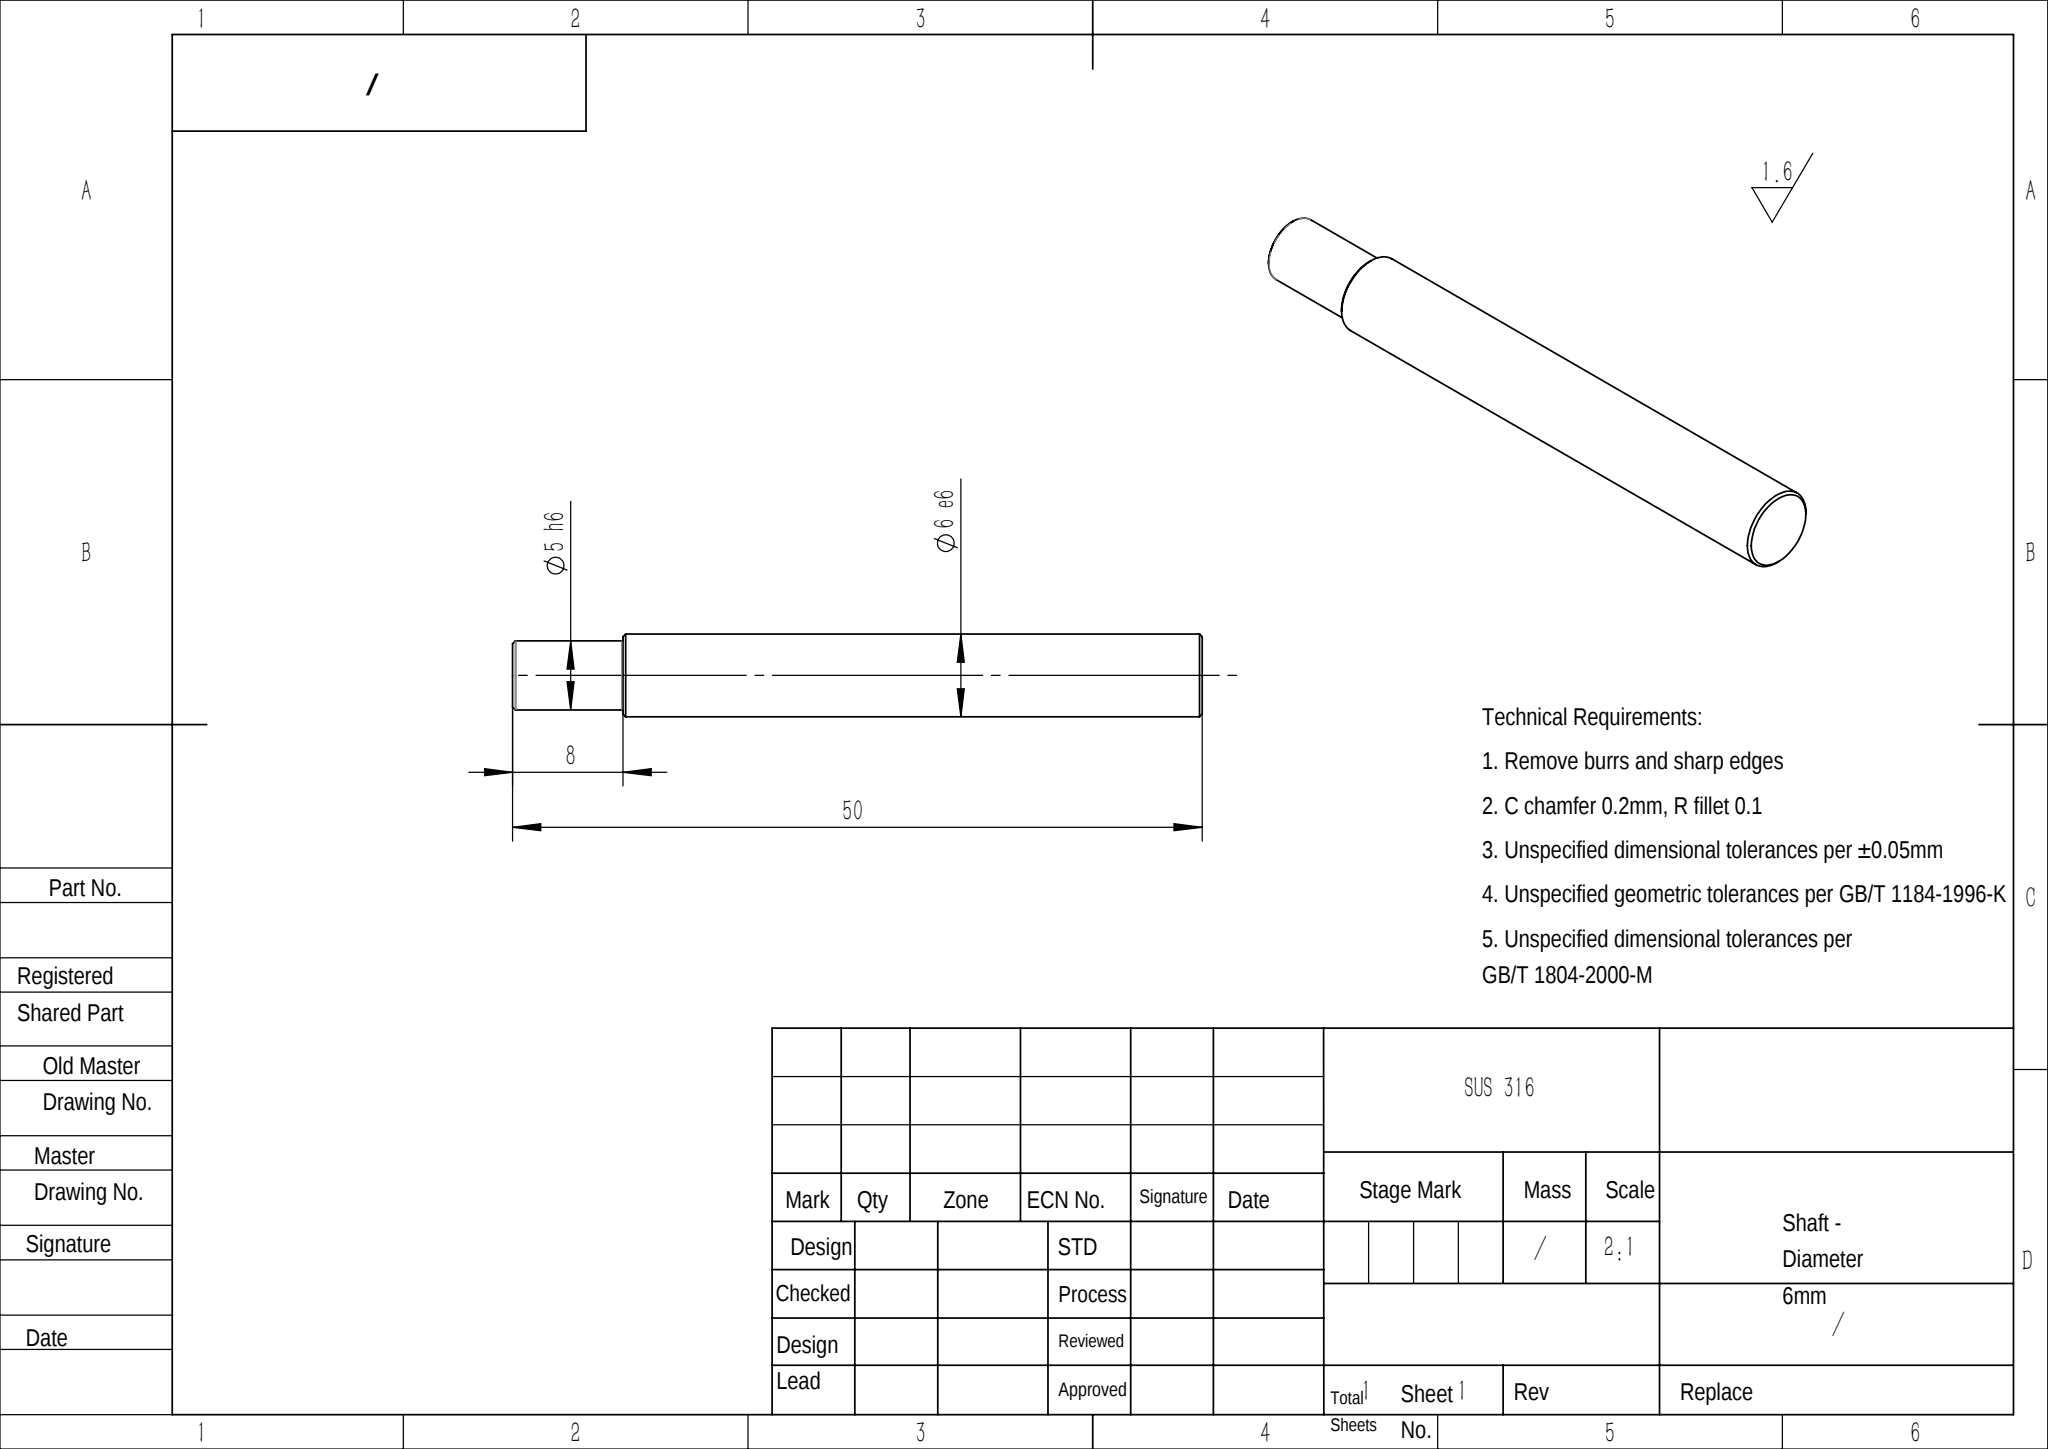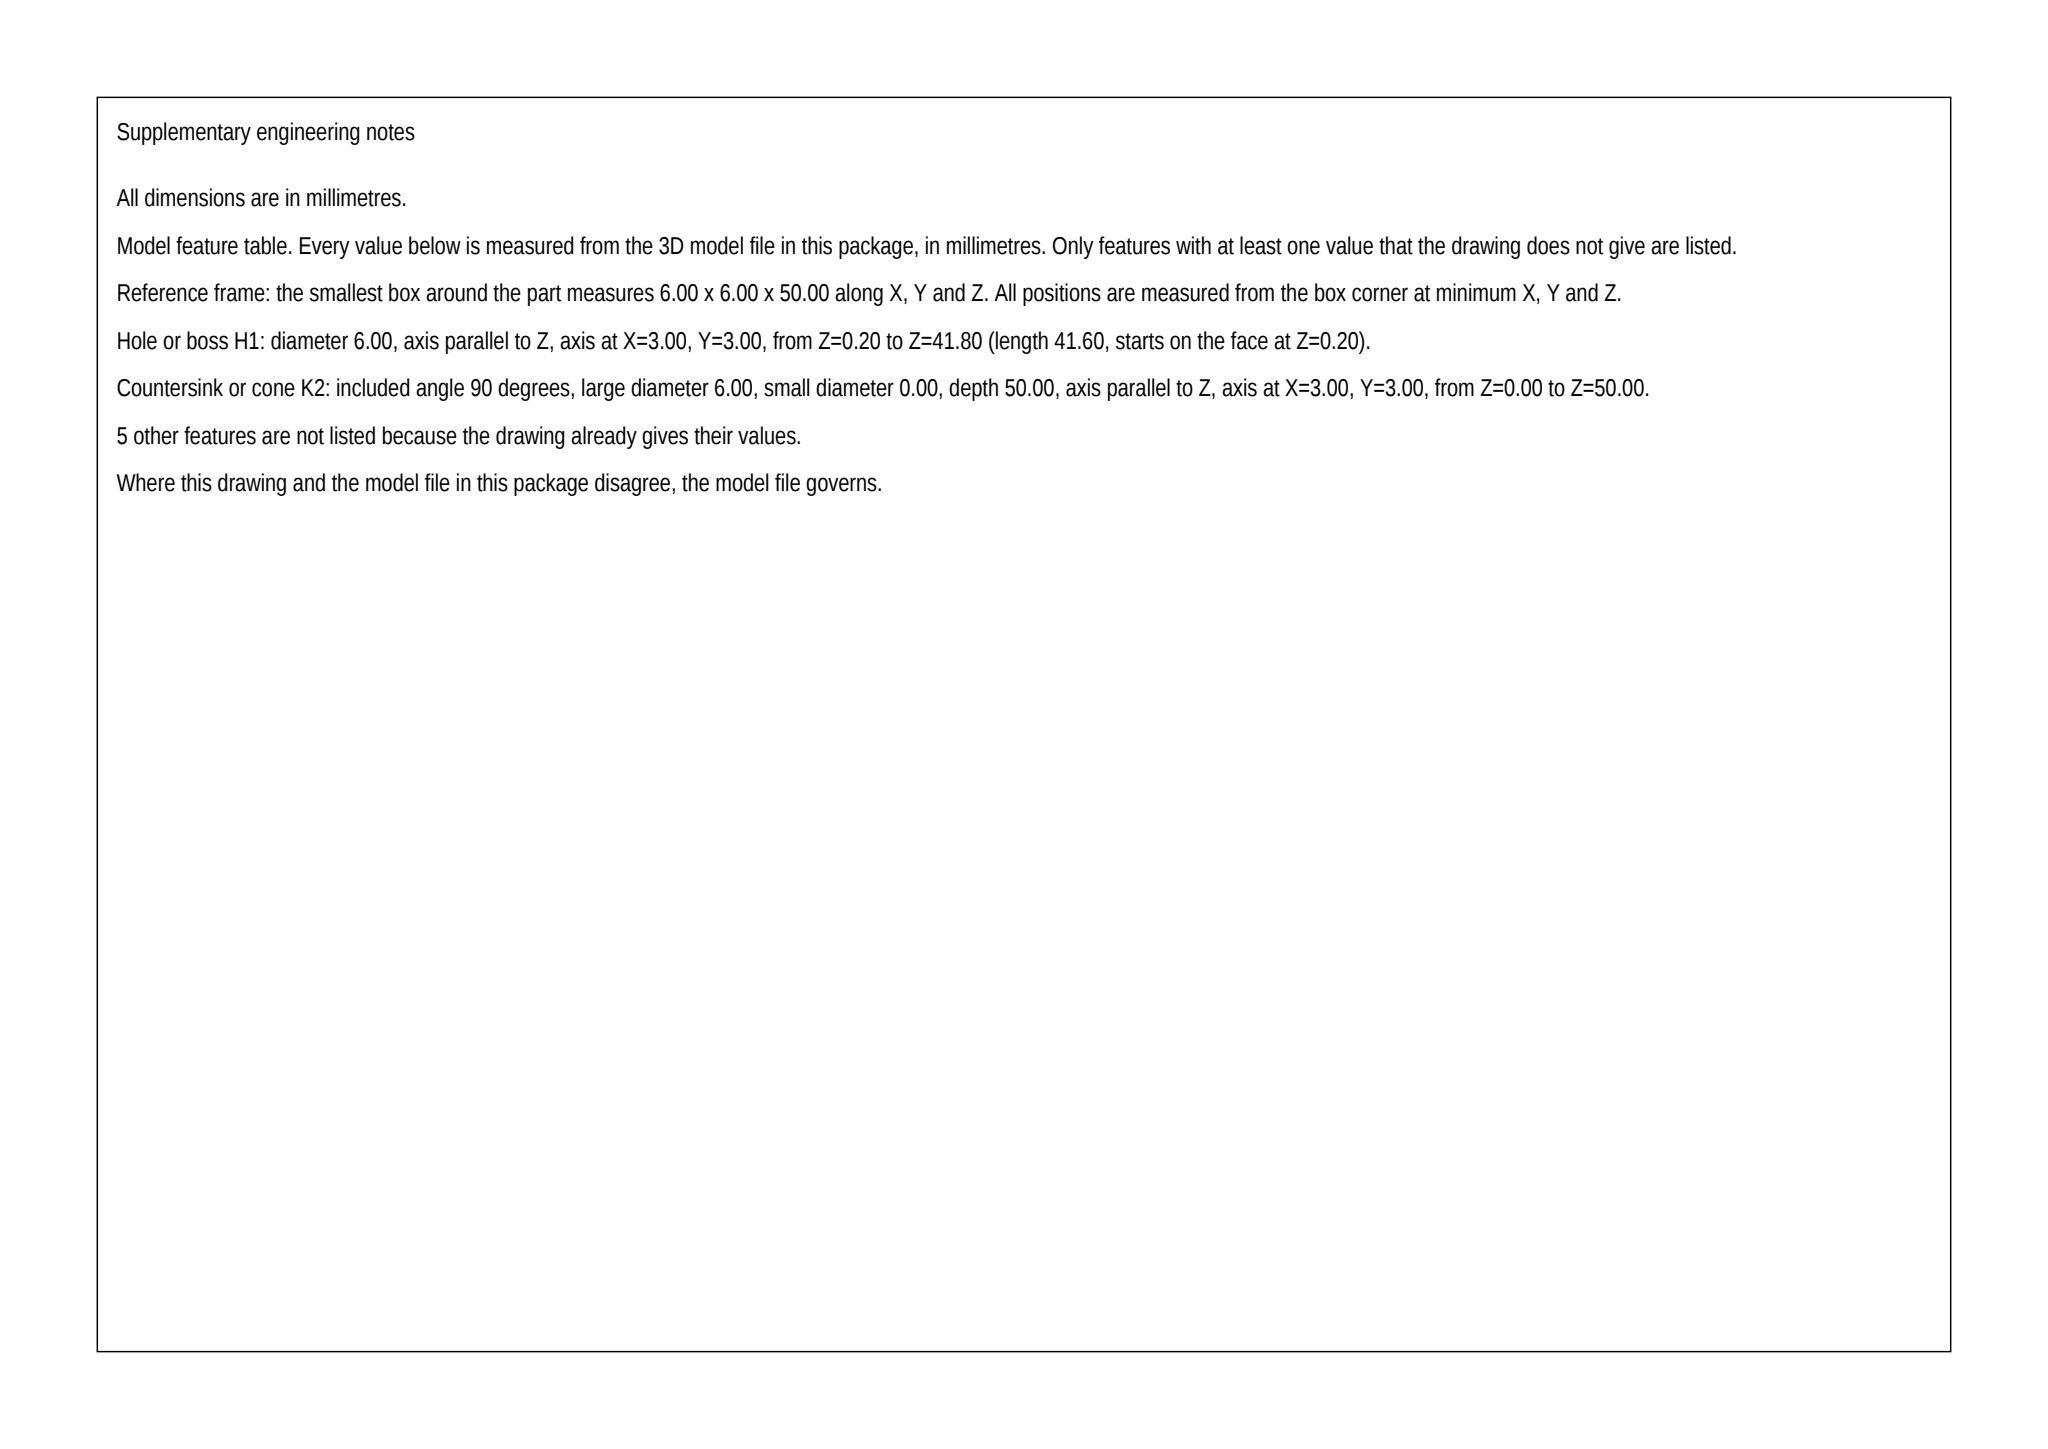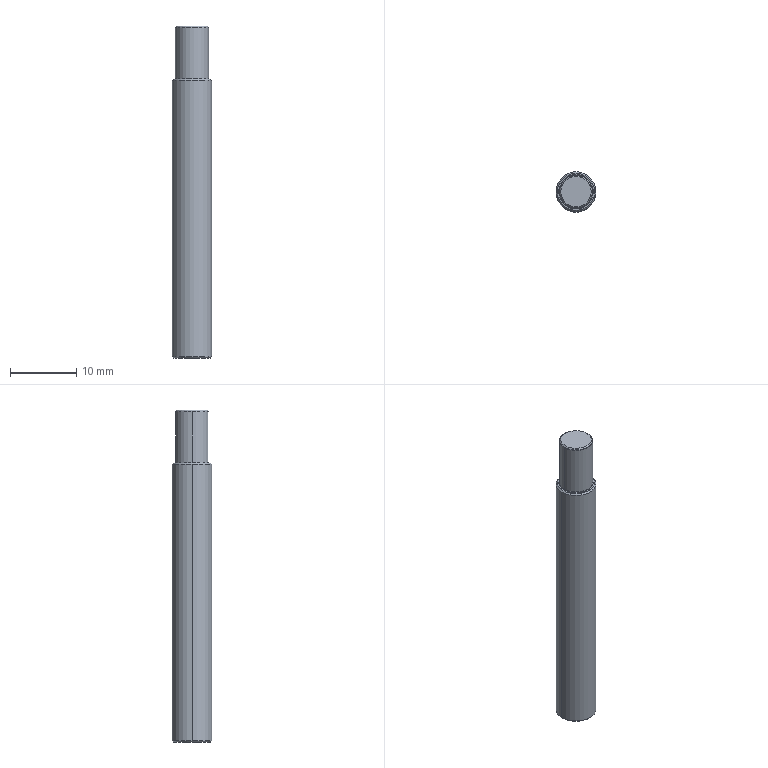Part | SolidWorks | mm | material SUS 316 | 1 solid | 17 faces | box 6 x 6 x 50 mm | volume 1344 mm3 | cone 6 | torus 4 | cylinder 4 | plane 3 | commonest cylinder face diameters 5 x2 6 x2
build123d program:
from build123d import *

# Parameters (mm, degrees)
SKETCH1_R           = 3
BOSS_EXTRUDE1_DEPTH = 50
CHAMFER1_SIZE       = 0.2
SKETCH2_R           = 3.9
SKETCH2_R_2         = 2.5
CUT_EXTRUDE1_DEPTH  = 8
CHAMFER2_SIZE       = 0.2
FILLET1_R           = 0.1


with BuildPart() as part:
    # Sketch1 → Boss-Extrude1 (new body)
    with BuildSketch(Plane.XY):
        Circle(SKETCH1_R)
    extrude(amount=BOSS_EXTRUDE1_DEPTH)

    # Chamfer1
    chamfer1_edges = [part.edges().sort_by_distance(p)[0] for p in [
        (-3, 0, 0),
        (-3, 0, 50),
    ]]
    chamfer(chamfer1_edges, length=CHAMFER1_SIZE)

    # Sketch2 → Cut-Extrude1 (cut)
    with BuildSketch(Plane.XY.offset(50)):
        Circle(SKETCH2_R)
        Circle(SKETCH2_R_2, mode=Mode.SUBTRACT)
    extrude(amount=-CUT_EXTRUDE1_DEPTH, mode=Mode.SUBTRACT)

    # Chamfer2
    chamfer2_edges = [part.edges().sort_by_distance(p)[0] for p in [
        (-3, 0, 42),
        (-2.5, 0, 50),
    ]]
    chamfer(chamfer2_edges, length=CHAMFER2_SIZE)

    # Fillet1
    fillet1_edges = [part.edges().sort_by_distance(p)[0] for p in [
        (-2.5, 0, 42),
        (-2.5, 0, 49.8),
    ]]
    fillet(fillet1_edges, radius=FILLET1_R)


solid = part.part
STEP:
#1=CARTESIAN_POINT('',(-2.5,0.,49.759));
#2=VERTEX_POINT('',#1);
#3=CARTESIAN_POINT('',(2.5,0.,49.759));
#4=VERTEX_POINT('',#3);
#5=CARTESIAN_POINT('',(0.,0.,49.759));
#6=DIRECTION('',(0.,0.,-1.));
#7=DIRECTION('',(1.,0.,0.));
#8=AXIS2_PLACEMENT_3D('',#5,#6,#7);
#9=CIRCLE('',#8,2.5);
#10=EDGE_CURVE('',#2,#4,#9,.T.);
#11=ORIENTED_EDGE('',*,*,#10,.F.);
#12=CARTESIAN_POINT('',(-2.471,0.,49.829));
#13=VERTEX_POINT('',#12);
#14=CARTESIAN_POINT('',(-2.4,0.,49.759));
#15=DIRECTION('',(0.,1.,0.));
#16=DIRECTION('',(-1.,0.,0.));
#17=AXIS2_PLACEMENT_3D('',#14,#15,#16);
#18=CIRCLE('',#17,0.1);
#19=EDGE_CURVE('',#2,#13,#18,.T.);
#20=ORIENTED_EDGE('',*,*,#19,.T.);
#21=CARTESIAN_POINT('',(2.471,0.,49.829));
#22=VERTEX_POINT('',#21);
#23=CARTESIAN_POINT('',(0.,0.,49.829));
#24=DIRECTION('',(0.,0.,1.));
#25=DIRECTION('',(1.,0.,0.));
#26=AXIS2_PLACEMENT_3D('',#23,#24,#25);
#27=CIRCLE('',#26,2.471);
#28=EDGE_CURVE('',#22,#13,#27,.T.);
#29=ORIENTED_EDGE('',*,*,#28,.F.);
#30=CARTESIAN_POINT('',(2.4,0.,49.759));
#31=DIRECTION('',(0.,-1.,0.));
#32=DIRECTION('',(0.,0.,-1.));
#33=AXIS2_PLACEMENT_3D('',#30,#31,#32);
#34=CIRCLE('',#33,0.1);
#35=EDGE_CURVE('',#4,#22,#34,.T.);
#36=ORIENTED_EDGE('',*,*,#35,.F.);
#37=EDGE_LOOP('',(#11,#20,#29,#36));
#38=FACE_OUTER_BOUND('',#37,.T.);
#39=CARTESIAN_POINT('',(0.,0.,49.759));
#40=DIRECTION('',(0.,0.,1.));
#41=DIRECTION('',(1.,0.,0.));
#42=AXIS2_PLACEMENT_3D('',#39,#40,#41);
#43=TOROIDAL_SURFACE('',#42,2.4,0.1);
#44=ADVANCED_FACE('',(#38),#43,.T.);
#45=CARTESIAN_POINT('',(-2.5,0.,42.1));
#46=VERTEX_POINT('',#45);
#47=CARTESIAN_POINT('',(2.5,0.,42.1));
#48=VERTEX_POINT('',#47);
#49=CARTESIAN_POINT('',(0.,0.,42.1));
#50=DIRECTION('',(0.,0.,1.));
#51=DIRECTION('',(1.,0.,0.));
#52=AXIS2_PLACEMENT_3D('',#49,#50,#51);
#53=CIRCLE('',#52,2.5);
#54=EDGE_CURVE('',#46,#48,#53,.T.);
#55=ORIENTED_EDGE('',*,*,#54,.F.);
#56=CARTESIAN_POINT('',(-2.6,0.,42.));
#57=VERTEX_POINT('',#56);
#58=CARTESIAN_POINT('',(-2.6,0.,42.1));
#59=DIRECTION('',(0.,1.,0.));
#60=DIRECTION('',(-1.,0.,0.));
#61=AXIS2_PLACEMENT_3D('',#58,#59,#60);
#62=CIRCLE('',#61,0.1);
#63=EDGE_CURVE('',#46,#57,#62,.T.);
#64=ORIENTED_EDGE('',*,*,#63,.T.);
#65=CARTESIAN_POINT('',(2.6,0.,42.));
#66=VERTEX_POINT('',#65);
#67=CARTESIAN_POINT('',(0.,0.,42.));
#68=DIRECTION('',(0.,0.,-1.));
#69=DIRECTION('',(1.,0.,0.));
#70=AXIS2_PLACEMENT_3D('',#67,#68,#69);
#71=CIRCLE('',#70,2.6);
#72=EDGE_CURVE('',#66,#57,#71,.T.);
#73=ORIENTED_EDGE('',*,*,#72,.F.);
#74=CARTESIAN_POINT('',(2.6,0.,42.1));
#75=DIRECTION('',(0.,-1.,0.));
#76=DIRECTION('',(0.,0.,-1.));
#77=AXIS2_PLACEMENT_3D('',#74,#75,#76);
#78=CIRCLE('',#77,0.1);
#79=EDGE_CURVE('',#48,#66,#78,.T.);
#80=ORIENTED_EDGE('',*,*,#79,.F.);
#81=EDGE_LOOP('',(#55,#64,#73,#80));
#82=FACE_OUTER_BOUND('',#81,.T.);
#83=CARTESIAN_POINT('',(0.,0.,42.1));
#84=DIRECTION('',(0.,0.,1.));
#85=DIRECTION('',(1.,0.,0.));
#86=AXIS2_PLACEMENT_3D('',#83,#84,#85);
#87=TOROIDAL_SURFACE('',#86,2.6,0.1);
#88=ADVANCED_FACE('',(#82),#87,.F.);
#89=CARTESIAN_POINT('',(2.3,0.,50.));
#90=VERTEX_POINT('',#89);
#91=CARTESIAN_POINT('',(-2.3,0.,50.));
#92=VERTEX_POINT('',#91);
#93=CARTESIAN_POINT('',(0.,0.,50.));
#94=DIRECTION('',(0.,0.,1.));
#95=DIRECTION('',(1.,0.,0.));
#96=AXIS2_PLACEMENT_3D('',#93,#94,#95);
#97=CIRCLE('',#96,2.3);
#98=EDGE_CURVE('',#90,#92,#97,.T.);
#99=ORIENTED_EDGE('',*,*,#98,.F.);
#100=CARTESIAN_POINT('',(2.3,0.,50.));
#101=DIRECTION('',(0.7071,0.,-0.7071));
#102=VECTOR('',#101,1000.);
#103=LINE('',#100,#102);
#104=EDGE_CURVE('',#90,#22,#103,.T.);
#105=ORIENTED_EDGE('',*,*,#104,.T.);
#106=ORIENTED_EDGE('',*,*,#28,.T.);
#107=CARTESIAN_POINT('',(-2.3,0.,50.));
#108=DIRECTION('',(-0.7071,0.,-0.7071));
#109=VECTOR('',#108,1000.);
#110=LINE('',#107,#109);
#111=EDGE_CURVE('',#92,#13,#110,.T.);
#112=ORIENTED_EDGE('',*,*,#111,.F.);
#113=EDGE_LOOP('',(#99,#105,#106,#112));
#114=FACE_OUTER_BOUND('',#113,.T.);
#115=CARTESIAN_POINT('',(0.,0.,50.));
#116=DIRECTION('',(0.,0.,-1.));
#117=DIRECTION('',(-1.,0.,0.));
#118=AXIS2_PLACEMENT_3D('',#115,#116,#117);
#119=CONICAL_SURFACE('',#118,2.3,0.7854);
#120=ADVANCED_FACE('',(#114),#119,.T.);
#121=CARTESIAN_POINT('',(2.8,0.,42.));
#122=VERTEX_POINT('',#121);
#123=CARTESIAN_POINT('',(-2.8,0.,42.));
#124=VERTEX_POINT('',#123);
#125=CARTESIAN_POINT('',(0.,0.,42.));
#126=DIRECTION('',(0.,0.,1.));
#127=DIRECTION('',(1.,0.,0.));
#128=AXIS2_PLACEMENT_3D('',#125,#126,#127);
#129=CIRCLE('',#128,2.8);
#130=EDGE_CURVE('',#122,#124,#129,.T.);
#131=ORIENTED_EDGE('',*,*,#130,.F.);
#132=CARTESIAN_POINT('',(3.,0.,41.8));
#133=VERTEX_POINT('',#132);
#134=CARTESIAN_POINT('',(2.8,0.,42.));
#135=DIRECTION('',(0.7071,0.,-0.7071));
#136=VECTOR('',#135,1000.);
#137=LINE('',#134,#136);
#138=EDGE_CURVE('',#122,#133,#137,.T.);
#139=ORIENTED_EDGE('',*,*,#138,.T.);
#140=CARTESIAN_POINT('',(-3.,0.,41.8));
#141=VERTEX_POINT('',#140);
#142=CARTESIAN_POINT('',(0.,0.,41.8));
#143=DIRECTION('',(0.,0.,-1.));
#144=DIRECTION('',(1.,0.,0.));
#145=AXIS2_PLACEMENT_3D('',#142,#143,#144);
#146=CIRCLE('',#145,3.);
#147=EDGE_CURVE('',#141,#133,#146,.T.);
#148=ORIENTED_EDGE('',*,*,#147,.F.);
#149=CARTESIAN_POINT('',(-2.8,0.,42.));
#150=DIRECTION('',(-0.7071,0.,-0.7071));
#151=VECTOR('',#150,1000.);
#152=LINE('',#149,#151);
#153=EDGE_CURVE('',#124,#141,#152,.T.);
#154=ORIENTED_EDGE('',*,*,#153,.F.);
#155=EDGE_LOOP('',(#131,#139,#148,#154));
#156=FACE_OUTER_BOUND('',#155,.T.);
#157=CARTESIAN_POINT('',(0.,0.,42.));
#158=DIRECTION('',(0.,0.,-1.));
#159=DIRECTION('',(-1.,0.,0.));
#160=AXIS2_PLACEMENT_3D('',#157,#158,#159);
#161=CONICAL_SURFACE('',#160,2.8,0.7854);
#162=ADVANCED_FACE('',(#156),#161,.T.);
#163=CARTESIAN_POINT('',(0.,0.,42.1));
#164=DIRECTION('',(0.,0.,1.));
#165=DIRECTION('',(1.,0.,0.));
#166=AXIS2_PLACEMENT_3D('',#163,#164,#165);
#167=CIRCLE('',#166,2.5);
#168=EDGE_CURVE('',#48,#46,#167,.T.);
#169=ORIENTED_EDGE('',*,*,#168,.T.);
#170=CARTESIAN_POINT('',(-2.5,0.,42.));
#171=DIRECTION('',(0.,0.,1.));
#172=VECTOR('',#171,1000.);
#173=LINE('',#170,#172);
#174=EDGE_CURVE('',#46,#2,#173,.T.);
#175=ORIENTED_EDGE('',*,*,#174,.T.);
#176=ORIENTED_EDGE('',*,*,#10,.T.);
#177=CARTESIAN_POINT('',(2.5,0.,42.));
#178=DIRECTION('',(0.,0.,1.));
#179=VECTOR('',#178,1000.);
#180=LINE('',#177,#179);
#181=EDGE_CURVE('',#48,#4,#180,.T.);
#182=ORIENTED_EDGE('',*,*,#181,.F.);
#183=EDGE_LOOP('',(#169,#175,#176,#182));
#184=FACE_OUTER_BOUND('',#183,.T.);
#185=CARTESIAN_POINT('',(0.,0.,42.));
#186=DIRECTION('',(0.,0.,1.));
#187=DIRECTION('',(1.,0.,0.));
#188=AXIS2_PLACEMENT_3D('',#185,#186,#187);
#189=CYLINDRICAL_SURFACE('',#188,2.5);
#190=ADVANCED_FACE('',(#184),#189,.T.);
#191=CARTESIAN_POINT('',(-2.8,0.,0.));
#192=VERTEX_POINT('',#191);
#193=CARTESIAN_POINT('',(2.8,0.,0.));
#194=VERTEX_POINT('',#193);
#195=CARTESIAN_POINT('',(0.,0.,0.));
#196=DIRECTION('',(0.,0.,-1.));
#197=DIRECTION('',(1.,0.,0.));
#198=AXIS2_PLACEMENT_3D('',#195,#196,#197);
#199=CIRCLE('',#198,2.8);
#200=EDGE_CURVE('',#192,#194,#199,.T.);
#201=ORIENTED_EDGE('',*,*,#200,.F.);
#202=CARTESIAN_POINT('',(-3.,0.,0.2));
#203=VERTEX_POINT('',#202);
#204=CARTESIAN_POINT('',(-3.,0.,0.2));
#205=DIRECTION('',(-0.7071,0.,0.7071));
#206=VECTOR('',#205,1000.);
#207=LINE('',#204,#206);
#208=EDGE_CURVE('',#192,#203,#207,.T.);
#209=ORIENTED_EDGE('',*,*,#208,.T.);
#210=CARTESIAN_POINT('',(3.,0.,0.2));
#211=VERTEX_POINT('',#210);
#212=CARTESIAN_POINT('',(0.,0.,0.2));
#213=DIRECTION('',(0.,0.,1.));
#214=DIRECTION('',(1.,0.,0.));
#215=AXIS2_PLACEMENT_3D('',#212,#213,#214);
#216=CIRCLE('',#215,3.);
#217=EDGE_CURVE('',#211,#203,#216,.T.);
#218=ORIENTED_EDGE('',*,*,#217,.F.);
#219=CARTESIAN_POINT('',(3.,0.,0.2));
#220=DIRECTION('',(0.7071,0.,0.7071));
#221=VECTOR('',#220,1000.);
#222=LINE('',#219,#221);
#223=EDGE_CURVE('',#194,#211,#222,.T.);
#224=ORIENTED_EDGE('',*,*,#223,.F.);
#225=EDGE_LOOP('',(#201,#209,#218,#224));
#226=FACE_OUTER_BOUND('',#225,.T.);
#227=CARTESIAN_POINT('',(0.,0.,0.2));
#228=DIRECTION('',(0.,0.,1.));
#229=DIRECTION('',(1.,0.,0.));
#230=AXIS2_PLACEMENT_3D('',#227,#228,#229);
#231=CONICAL_SURFACE('',#230,3.,0.7854);
#232=ADVANCED_FACE('',(#226),#231,.T.);
#233=ORIENTED_EDGE('',*,*,#147,.T.);
#234=CARTESIAN_POINT('',(3.,0.,50.));
#235=DIRECTION('',(0.,0.,-1.));
#236=VECTOR('',#235,1000.);
#237=LINE('',#234,#236);
#238=EDGE_CURVE('',#133,#211,#237,.T.);
#239=ORIENTED_EDGE('',*,*,#238,.T.);
#240=ORIENTED_EDGE('',*,*,#217,.T.);
#241=CARTESIAN_POINT('',(-3.,0.,50.));
#242=DIRECTION('',(0.,0.,-1.));
#243=VECTOR('',#242,1000.);
#244=LINE('',#241,#243);
#245=EDGE_CURVE('',#141,#203,#244,.T.);
#246=ORIENTED_EDGE('',*,*,#245,.F.);
#247=EDGE_LOOP('',(#233,#239,#240,#246));
#248=FACE_OUTER_BOUND('',#247,.T.);
#249=CARTESIAN_POINT('',(0.,0.,50.));
#250=DIRECTION('',(0.,0.,-1.));
#251=DIRECTION('',(-1.,0.,0.));
#252=AXIS2_PLACEMENT_3D('',#249,#250,#251);
#253=CYLINDRICAL_SURFACE('',#252,3.);
#254=ADVANCED_FACE('',(#248),#253,.T.);
#255=ORIENTED_EDGE('',*,*,#238,.F.);
#256=CARTESIAN_POINT('',(0.,0.,41.8));
#257=DIRECTION('',(0.,0.,-1.));
#258=DIRECTION('',(1.,0.,0.));
#259=AXIS2_PLACEMENT_3D('',#256,#257,#258);
#260=CIRCLE('',#259,3.);
#261=EDGE_CURVE('',#133,#141,#260,.T.);
#262=ORIENTED_EDGE('',*,*,#261,.T.);
#263=ORIENTED_EDGE('',*,*,#245,.T.);
#264=CARTESIAN_POINT('',(0.,0.,0.2));
#265=DIRECTION('',(0.,0.,1.));
#266=DIRECTION('',(1.,0.,0.));
#267=AXIS2_PLACEMENT_3D('',#264,#265,#266);
#268=CIRCLE('',#267,3.);
#269=EDGE_CURVE('',#203,#211,#268,.T.);
#270=ORIENTED_EDGE('',*,*,#269,.T.);
#271=EDGE_LOOP('',(#255,#262,#263,#270));
#272=FACE_OUTER_BOUND('',#271,.T.);
#273=CARTESIAN_POINT('',(0.,0.,50.));
#274=DIRECTION('',(0.,0.,-1.));
#275=DIRECTION('',(-1.,0.,0.));
#276=AXIS2_PLACEMENT_3D('',#273,#274,#275);
#277=CYLINDRICAL_SURFACE('',#276,3.);
#278=ADVANCED_FACE('',(#272),#277,.T.);
#279=CARTESIAN_POINT('',(0.,0.,0.));
#280=DIRECTION('',(0.,0.,-1.));
#281=DIRECTION('',(1.,0.,0.));
#282=AXIS2_PLACEMENT_3D('',#279,#280,#281);
#283=CIRCLE('',#282,2.8);
#284=EDGE_CURVE('',#194,#192,#283,.T.);
#285=ORIENTED_EDGE('',*,*,#284,.T.);
#286=ORIENTED_EDGE('',*,*,#200,.T.);
#287=EDGE_LOOP('',(#285,#286));
#288=FACE_OUTER_BOUND('',#287,.T.);
#289=CARTESIAN_POINT('',(0.,0.,0.));
#290=DIRECTION('',(0.,0.,1.));
#291=DIRECTION('',(1.,0.,0.));
#292=AXIS2_PLACEMENT_3D('',#289,#290,#291);
#293=PLANE('',#292);
#294=ADVANCED_FACE('',(#288),#293,.F.);
#295=ORIENTED_EDGE('',*,*,#208,.F.);
#296=ORIENTED_EDGE('',*,*,#284,.F.);
#297=ORIENTED_EDGE('',*,*,#223,.T.);
#298=ORIENTED_EDGE('',*,*,#269,.F.);
#299=EDGE_LOOP('',(#295,#296,#297,#298));
#300=FACE_OUTER_BOUND('',#299,.T.);
#301=CARTESIAN_POINT('',(0.,0.,0.2));
#302=DIRECTION('',(0.,0.,1.));
#303=DIRECTION('',(1.,0.,0.));
#304=AXIS2_PLACEMENT_3D('',#301,#302,#303);
#305=CONICAL_SURFACE('',#304,3.,0.7854);
#306=ADVANCED_FACE('',(#300),#305,.T.);
#307=ORIENTED_EDGE('',*,*,#72,.T.);
#308=CARTESIAN_POINT('',(0.,0.,42.));
#309=DIRECTION('',(0.,0.,-1.));
#310=DIRECTION('',(1.,0.,0.));
#311=AXIS2_PLACEMENT_3D('',#308,#309,#310);
#312=CIRCLE('',#311,2.6);
#313=EDGE_CURVE('',#57,#66,#312,.T.);
#314=ORIENTED_EDGE('',*,*,#313,.T.);
#315=EDGE_LOOP('',(#307,#314));
#316=FACE_BOUND('',#315,.T.);
#317=CARTESIAN_POINT('',(0.,0.,42.));
#318=DIRECTION('',(0.,0.,1.));
#319=DIRECTION('',(1.,0.,0.));
#320=AXIS2_PLACEMENT_3D('',#317,#318,#319);
#321=CIRCLE('',#320,2.8);
#322=EDGE_CURVE('',#124,#122,#321,.T.);
#323=ORIENTED_EDGE('',*,*,#322,.T.);
#324=ORIENTED_EDGE('',*,*,#130,.T.);
#325=EDGE_LOOP('',(#323,#324));
#326=FACE_OUTER_BOUND('',#325,.T.);
#327=CARTESIAN_POINT('',(0.,0.,42.));
#328=DIRECTION('',(0.,0.,1.));
#329=DIRECTION('',(1.,0.,0.));
#330=AXIS2_PLACEMENT_3D('',#327,#328,#329);
#331=PLANE('',#330);
#332=ADVANCED_FACE('',(#316,#326),#331,.T.);
#333=ORIENTED_EDGE('',*,*,#174,.F.);
#334=ORIENTED_EDGE('',*,*,#54,.T.);
#335=ORIENTED_EDGE('',*,*,#181,.T.);
#336=CARTESIAN_POINT('',(0.,0.,49.759));
#337=DIRECTION('',(0.,0.,-1.));
#338=DIRECTION('',(1.,0.,0.));
#339=AXIS2_PLACEMENT_3D('',#336,#337,#338);
#340=CIRCLE('',#339,2.5);
#341=EDGE_CURVE('',#4,#2,#340,.T.);
#342=ORIENTED_EDGE('',*,*,#341,.T.);
#343=EDGE_LOOP('',(#333,#334,#335,#342));
#344=FACE_OUTER_BOUND('',#343,.T.);
#345=CARTESIAN_POINT('',(0.,0.,42.));
#346=DIRECTION('',(0.,0.,1.));
#347=DIRECTION('',(1.,0.,0.));
#348=AXIS2_PLACEMENT_3D('',#345,#346,#347);
#349=CYLINDRICAL_SURFACE('',#348,2.5);
#350=ADVANCED_FACE('',(#344),#349,.T.);
#351=CARTESIAN_POINT('',(0.,0.,50.));
#352=DIRECTION('',(0.,0.,1.));
#353=DIRECTION('',(1.,0.,0.));
#354=AXIS2_PLACEMENT_3D('',#351,#352,#353);
#355=CIRCLE('',#354,2.3);
#356=EDGE_CURVE('',#92,#90,#355,.T.);
#357=ORIENTED_EDGE('',*,*,#356,.T.);
#358=ORIENTED_EDGE('',*,*,#98,.T.);
#359=EDGE_LOOP('',(#357,#358));
#360=FACE_OUTER_BOUND('',#359,.T.);
#361=CARTESIAN_POINT('',(0.,0.,50.));
#362=DIRECTION('',(0.,0.,1.));
#363=DIRECTION('',(1.,0.,0.));
#364=AXIS2_PLACEMENT_3D('',#361,#362,#363);
#365=PLANE('',#364);
#366=ADVANCED_FACE('',(#360),#365,.T.);
#367=ORIENTED_EDGE('',*,*,#138,.F.);
#368=ORIENTED_EDGE('',*,*,#322,.F.);
#369=ORIENTED_EDGE('',*,*,#153,.T.);
#370=ORIENTED_EDGE('',*,*,#261,.F.);
#371=EDGE_LOOP('',(#367,#368,#369,#370));
#372=FACE_OUTER_BOUND('',#371,.T.);
#373=CARTESIAN_POINT('',(0.,0.,42.));
#374=DIRECTION('',(0.,0.,-1.));
#375=DIRECTION('',(-1.,0.,0.));
#376=AXIS2_PLACEMENT_3D('',#373,#374,#375);
#377=CONICAL_SURFACE('',#376,2.8,0.7854);
#378=ADVANCED_FACE('',(#372),#377,.T.);
#379=ORIENTED_EDGE('',*,*,#104,.F.);
#380=ORIENTED_EDGE('',*,*,#356,.F.);
#381=ORIENTED_EDGE('',*,*,#111,.T.);
#382=CARTESIAN_POINT('',(0.,0.,49.829));
#383=DIRECTION('',(0.,0.,1.));
#384=DIRECTION('',(1.,0.,0.));
#385=AXIS2_PLACEMENT_3D('',#382,#383,#384);
#386=CIRCLE('',#385,2.471);
#387=EDGE_CURVE('',#13,#22,#386,.T.);
#388=ORIENTED_EDGE('',*,*,#387,.T.);
#389=EDGE_LOOP('',(#379,#380,#381,#388));
#390=FACE_OUTER_BOUND('',#389,.T.);
#391=CARTESIAN_POINT('',(0.,0.,50.));
#392=DIRECTION('',(0.,0.,-1.));
#393=DIRECTION('',(-1.,0.,0.));
#394=AXIS2_PLACEMENT_3D('',#391,#392,#393);
#395=CONICAL_SURFACE('',#394,2.3,0.7854);
#396=ADVANCED_FACE('',(#390),#395,.T.);
#397=ORIENTED_EDGE('',*,*,#63,.F.);
#398=ORIENTED_EDGE('',*,*,#168,.F.);
#399=ORIENTED_EDGE('',*,*,#79,.T.);
#400=ORIENTED_EDGE('',*,*,#313,.F.);
#401=EDGE_LOOP('',(#397,#398,#399,#400));
#402=FACE_OUTER_BOUND('',#401,.T.);
#403=CARTESIAN_POINT('',(0.,0.,42.1));
#404=DIRECTION('',(0.,0.,1.));
#405=DIRECTION('',(1.,0.,0.));
#406=AXIS2_PLACEMENT_3D('',#403,#404,#405);
#407=TOROIDAL_SURFACE('',#406,2.6,0.1);
#408=ADVANCED_FACE('',(#402),#407,.F.);
#409=ORIENTED_EDGE('',*,*,#19,.F.);
#410=ORIENTED_EDGE('',*,*,#341,.F.);
#411=ORIENTED_EDGE('',*,*,#35,.T.);
#412=ORIENTED_EDGE('',*,*,#387,.F.);
#413=EDGE_LOOP('',(#409,#410,#411,#412));
#414=FACE_OUTER_BOUND('',#413,.T.);
#415=CARTESIAN_POINT('',(0.,0.,49.759));
#416=DIRECTION('',(0.,0.,1.));
#417=DIRECTION('',(1.,0.,0.));
#418=AXIS2_PLACEMENT_3D('',#415,#416,#417);
#419=TOROIDAL_SURFACE('',#418,2.4,0.1);
#420=ADVANCED_FACE('',(#414),#419,.T.);
#421=CLOSED_SHELL('',(#44,#88,#120,#162,#190,#232,#254,#278,#294,#306,#332,#350,#366,#378,#396,#408,#420));
#422=MANIFOLD_SOLID_BREP('',#421);
#423=CARTESIAN_POINT('',(0.,0.,0.));
#424=DIRECTION('',(0.,0.,1.));
#425=DIRECTION('',(1.,0.,0.));
#426=AXIS2_PLACEMENT_3D('',#423,#424,#425);
#427=(LENGTH_UNIT()NAMED_UNIT(*)SI_UNIT(.MILLI.,.METRE.));
#428=UNCERTAINTY_MEASURE_WITH_UNIT(LENGTH_MEASURE(0.00001),#427,'','');
#429=(NAMED_UNIT(*)PLANE_ANGLE_UNIT()SI_UNIT($,.RADIAN.));
#430=(NAMED_UNIT(*)SI_UNIT($,.STERADIAN.)SOLID_ANGLE_UNIT());
#431=(GEOMETRIC_REPRESENTATION_CONTEXT(3)GLOBAL_UNCERTAINTY_ASSIGNED_CONTEXT((#428))GLOBAL_UNIT_ASSIGNED_CONTEXT((#427,#429,#430))REPRESENTATION_CONTEXT('',''));
#432=ADVANCED_BREP_SHAPE_REPRESENTATION('',(#422,#426),#431);